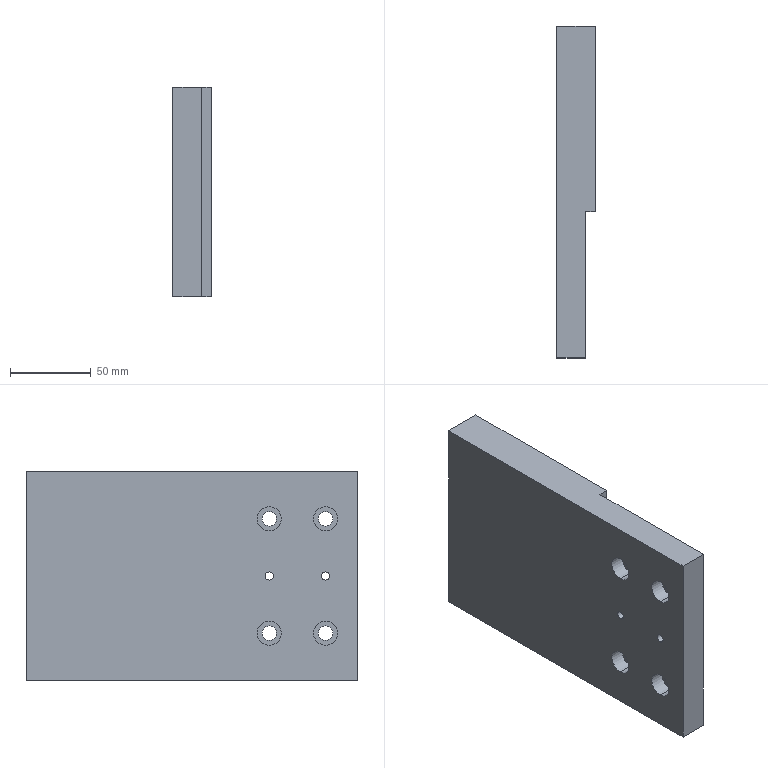Component | SolidWorks | SupportPlate-1 | 1 solid | 48 faces | box 24 x 206 x 130 mm | volume 559706 mm3 | cylinder 28 | plane 12 | cone 8 | commonest cylinder face diameters 5 x8 15 x8 9 x8 8 x4
build123d program:
from build123d import *

# Parameters (mm, degrees)
SKETCH1_W                                            = 130
SKETCH1_H                                            = 206
BOSS_EXTRUDE1_DEPTH                                  = 24
SKETCH2_W                                            = 6
SKETCH2_H                                            = 91
CUT_EXTRUDE1_DEPTH                                   = 164
SIZE_MM_DOWEL_PIN_HOLE_2_D                           = 5
SIZE_MM_DOWEL_PIN_HOLE_2_DEPTH                       = 36.25
SIZE_MM_DOWEL_PIN_HOLE_2_TIP                         = 1.502
HOLE_SIZE_ACCORDING_TO_HEXAGON_SOCKET_HE_D           = 9
HOLE_SIZE_ACCORDING_TO_HEXAGON_SOCKET_HE_DEPTH       = 36.25
HOLE_SIZE_ACCORDING_TO_HEXAGON_SOCKET_HE_CBORE_D     = 15
HOLE_SIZE_ACCORDING_TO_HEXAGON_SOCKET_HE_CBORE_DEPTH = 9
HOLE_SIZE_ACCORDING_TO_HEXAGON_SOCKET_HE_TIP         = 2.704
M8_TAPPED_HOLE1_D                                    = 8
M8_TAPPED_HOLE1_DEPTH                                = 19.75
M8_TAPPED_HOLE1_TIP                                  = 2.403
SIZE_MM_DOWEL_PIN_HOLE_2_2_D                         = 5
SIZE_MM_DOWEL_PIN_HOLE_2_2_DEPTH                     = 15
SIZE_MM_DOWEL_PIN_HOLE_2_2_TIP                       = 1.502


with BuildPart() as part:
    # Sketch1 → Boss-Extrude1 (new body)
    with BuildSketch(Plane.XY):
        with Locations((0, 103)):
            Rectangle(SKETCH1_W, SKETCH1_H)
    extrude(amount=-BOSS_EXTRUDE1_DEPTH)

    # Sketch2 → Cut-Extrude1 (cut)
    with BuildSketch(Plane(origin=(65, 0, 0), x_dir=(0, 0, -1), z_dir=(1, 0, 0))):
        with Locations((21, 45.5)):
            Rectangle(SKETCH2_W, SKETCH2_H)
    extrude(amount=-CUT_EXTRUDE1_DEPTH, mode=Mode.SUBTRACT)

    # Size mm Dowel Pin Hole 2
    with Locations(Plane.XY):
        with Locations((0, 20), (0, 55)):
            Hole(SIZE_MM_DOWEL_PIN_HOLE_2_D / 2, depth=SIZE_MM_DOWEL_PIN_HOLE_2_DEPTH)
            with Locations((0, 0, -(SIZE_MM_DOWEL_PIN_HOLE_2_DEPTH + SIZE_MM_DOWEL_PIN_HOLE_2_TIP / 2))):  # 118° drill point
                Cone(0, SIZE_MM_DOWEL_PIN_HOLE_2_D / 2, SIZE_MM_DOWEL_PIN_HOLE_2_TIP, mode=Mode.SUBTRACT)

    # Hole Size_According to_Hexagon Socket He
    with Locations(Plane.XY):
        with Locations((-35.5, 55), (35.5, 55), (-35.5, 20), (35.5, 20)):
            CounterBoreHole(HOLE_SIZE_ACCORDING_TO_HEXAGON_SOCKET_HE_D / 2, HOLE_SIZE_ACCORDING_TO_HEXAGON_SOCKET_HE_CBORE_D / 2, HOLE_SIZE_ACCORDING_TO_HEXAGON_SOCKET_HE_CBORE_DEPTH, depth=HOLE_SIZE_ACCORDING_TO_HEXAGON_SOCKET_HE_DEPTH)
            with Locations((0, 0, -(HOLE_SIZE_ACCORDING_TO_HEXAGON_SOCKET_HE_DEPTH + HOLE_SIZE_ACCORDING_TO_HEXAGON_SOCKET_HE_TIP / 2))):  # 118° drill point
                Cone(0, HOLE_SIZE_ACCORDING_TO_HEXAGON_SOCKET_HE_D / 2, HOLE_SIZE_ACCORDING_TO_HEXAGON_SOCKET_HE_TIP, mode=Mode.SUBTRACT)

    # M8 Tapped Hole1
    with Locations(Plane(origin=(0, 206, 0), x_dir=(1, 0, 0), z_dir=(0, 1, 0))):
        with Locations((-27.5, 12.362), (27.5, 12.362)):
            Hole(M8_TAPPED_HOLE1_D / 2, depth=M8_TAPPED_HOLE1_DEPTH)
            with Locations((0, 0, -(M8_TAPPED_HOLE1_DEPTH + M8_TAPPED_HOLE1_TIP / 2))):  # 118° drill point
                Cone(0, M8_TAPPED_HOLE1_D / 2, M8_TAPPED_HOLE1_TIP, mode=Mode.SUBTRACT)

    # Size mm Dowel Pin Hole 2_2
    with Locations(Plane(origin=(0, 206, 0), x_dir=(1, 0, 0), z_dir=(0, 1, 0))):
        with Locations((-48, 12.362), (48, 12.362)):
            Hole(SIZE_MM_DOWEL_PIN_HOLE_2_2_D / 2, depth=SIZE_MM_DOWEL_PIN_HOLE_2_2_DEPTH)
            with Locations((0, 0, -(SIZE_MM_DOWEL_PIN_HOLE_2_2_DEPTH + SIZE_MM_DOWEL_PIN_HOLE_2_2_TIP / 2))):  # 118° drill point
                Cone(0, SIZE_MM_DOWEL_PIN_HOLE_2_2_D / 2, SIZE_MM_DOWEL_PIN_HOLE_2_2_TIP, mode=Mode.SUBTRACT)


solid = part.part

# Placed as in the assembly
solid = solid.moved(Location((-165.862, 75, 0), (0, -90, 0)))